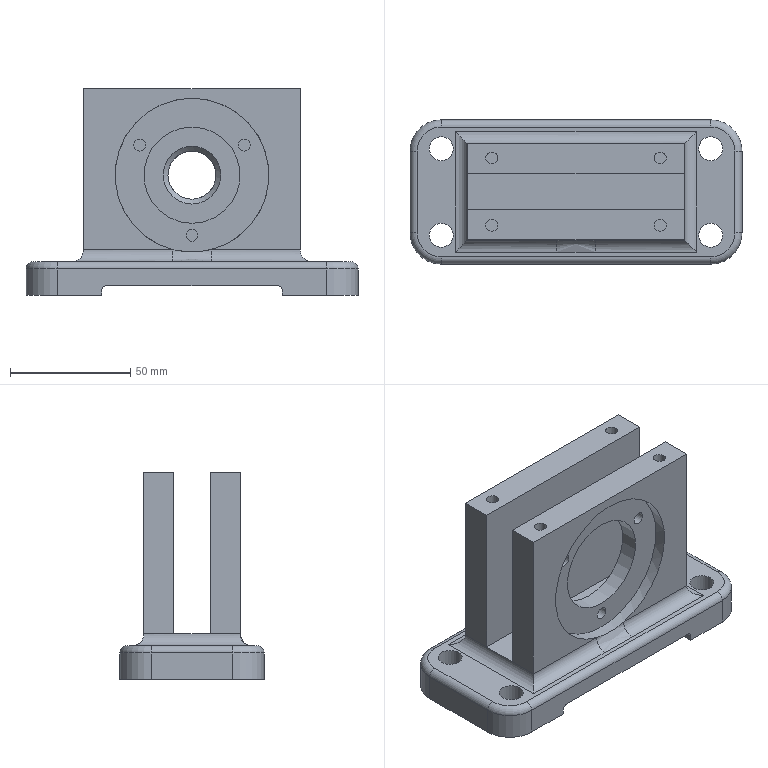Component | NX | HOUSING | 1 solid | 61 faces | volume 229486 mm3 | cylinder 29 | plane 26 | torus 4 | cone 1 | spline 1 | commonest cylinder face diameters 10 x9 5 x7 26 x4 6 x4 4 x2 40 x1 64 x1 20 x1